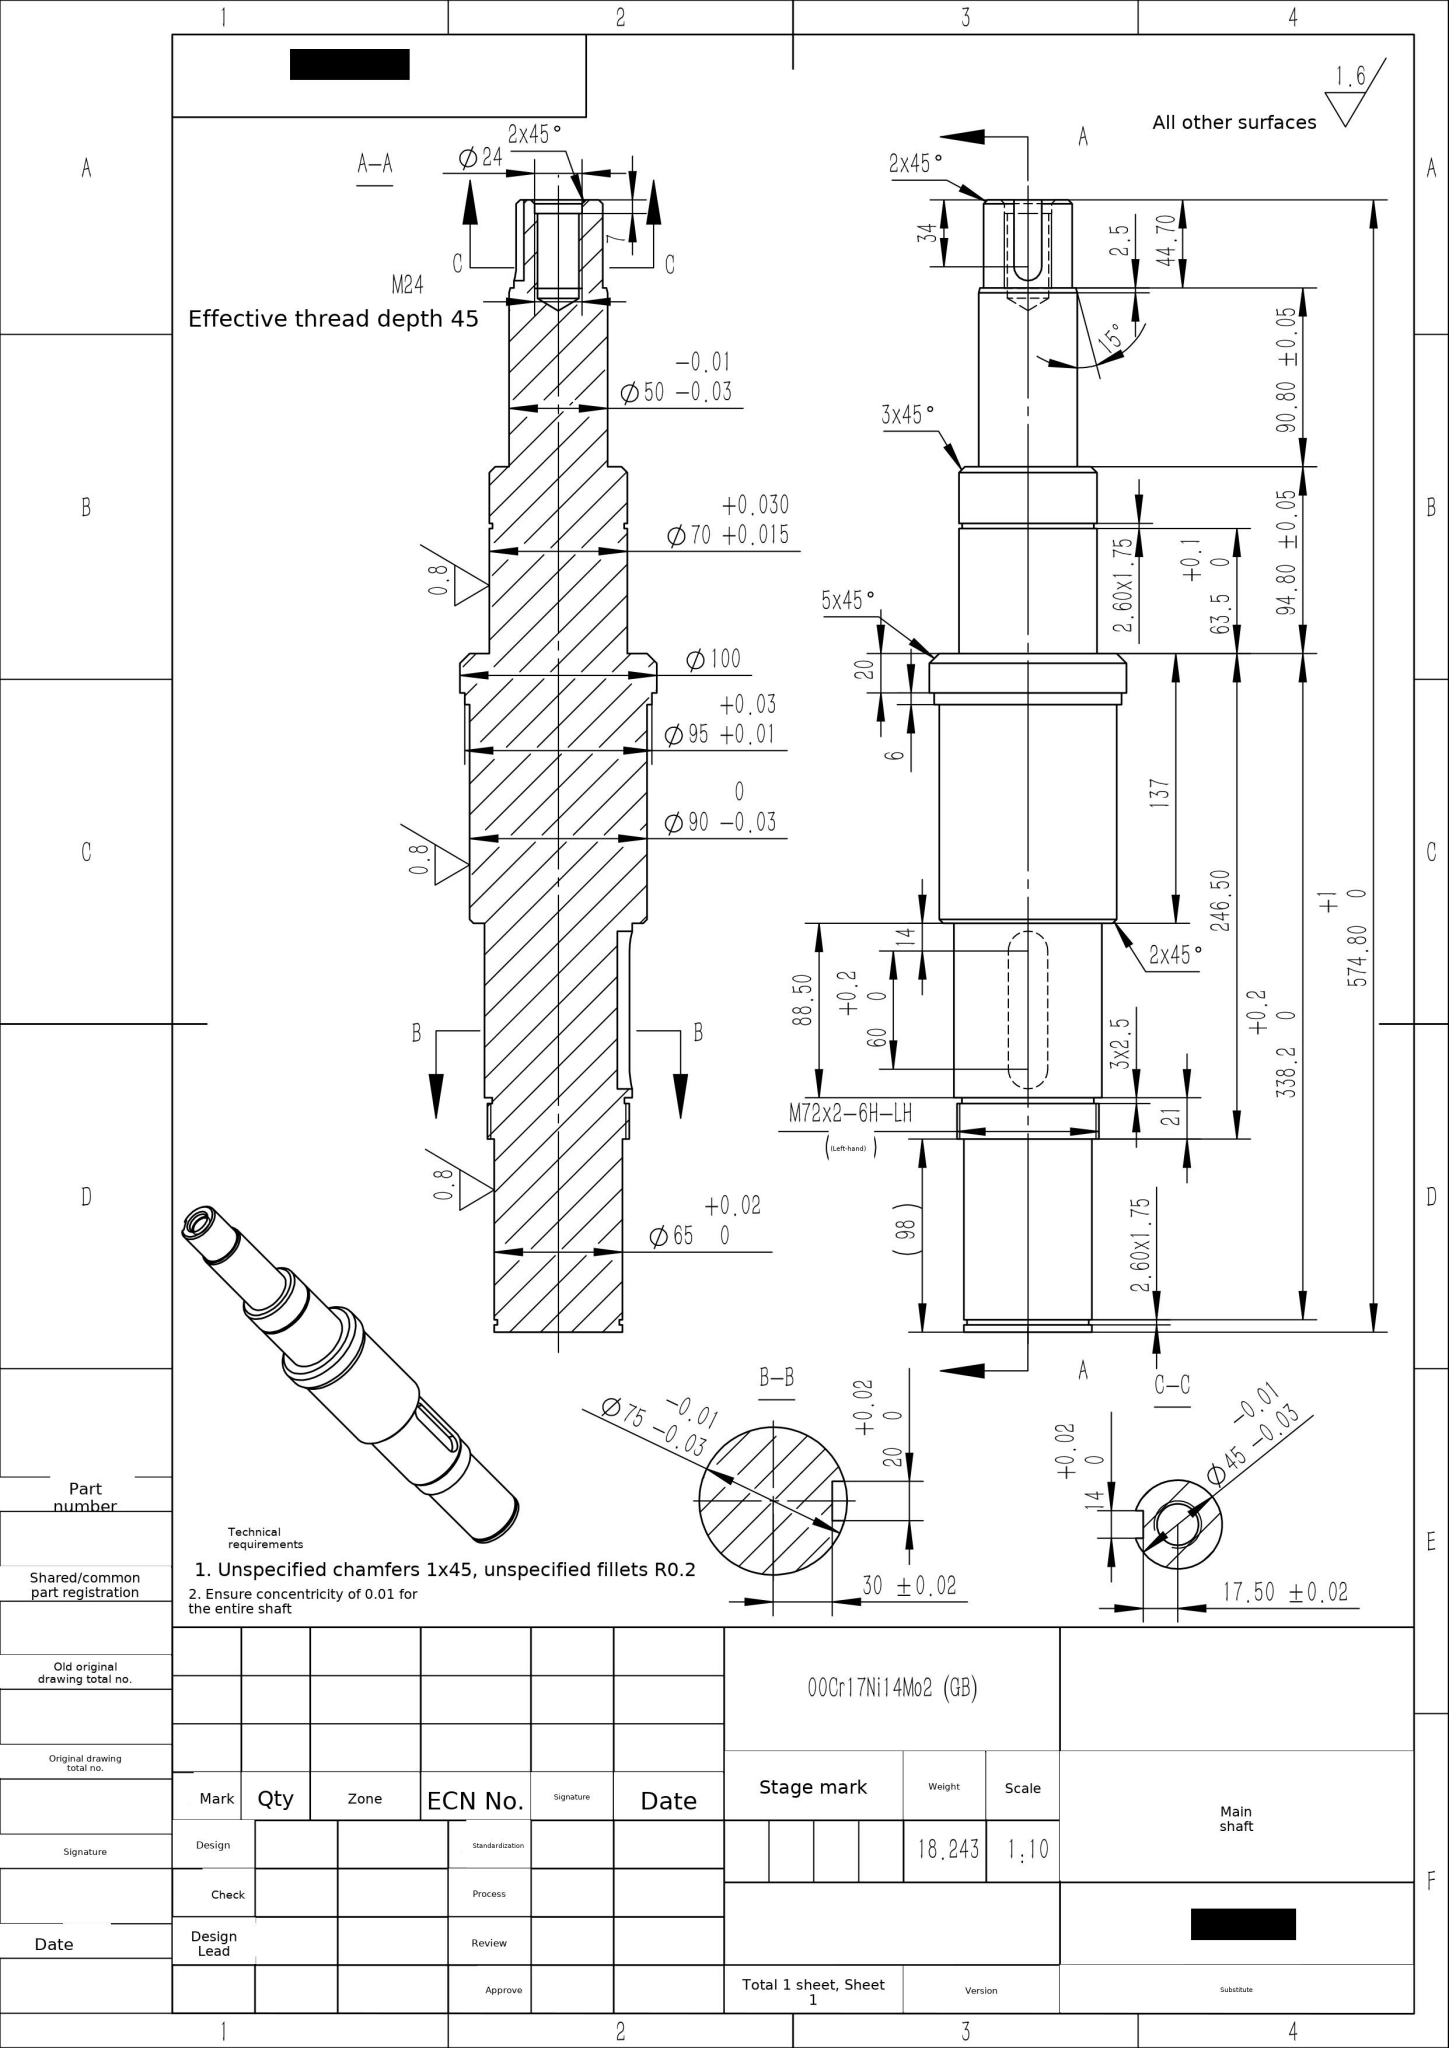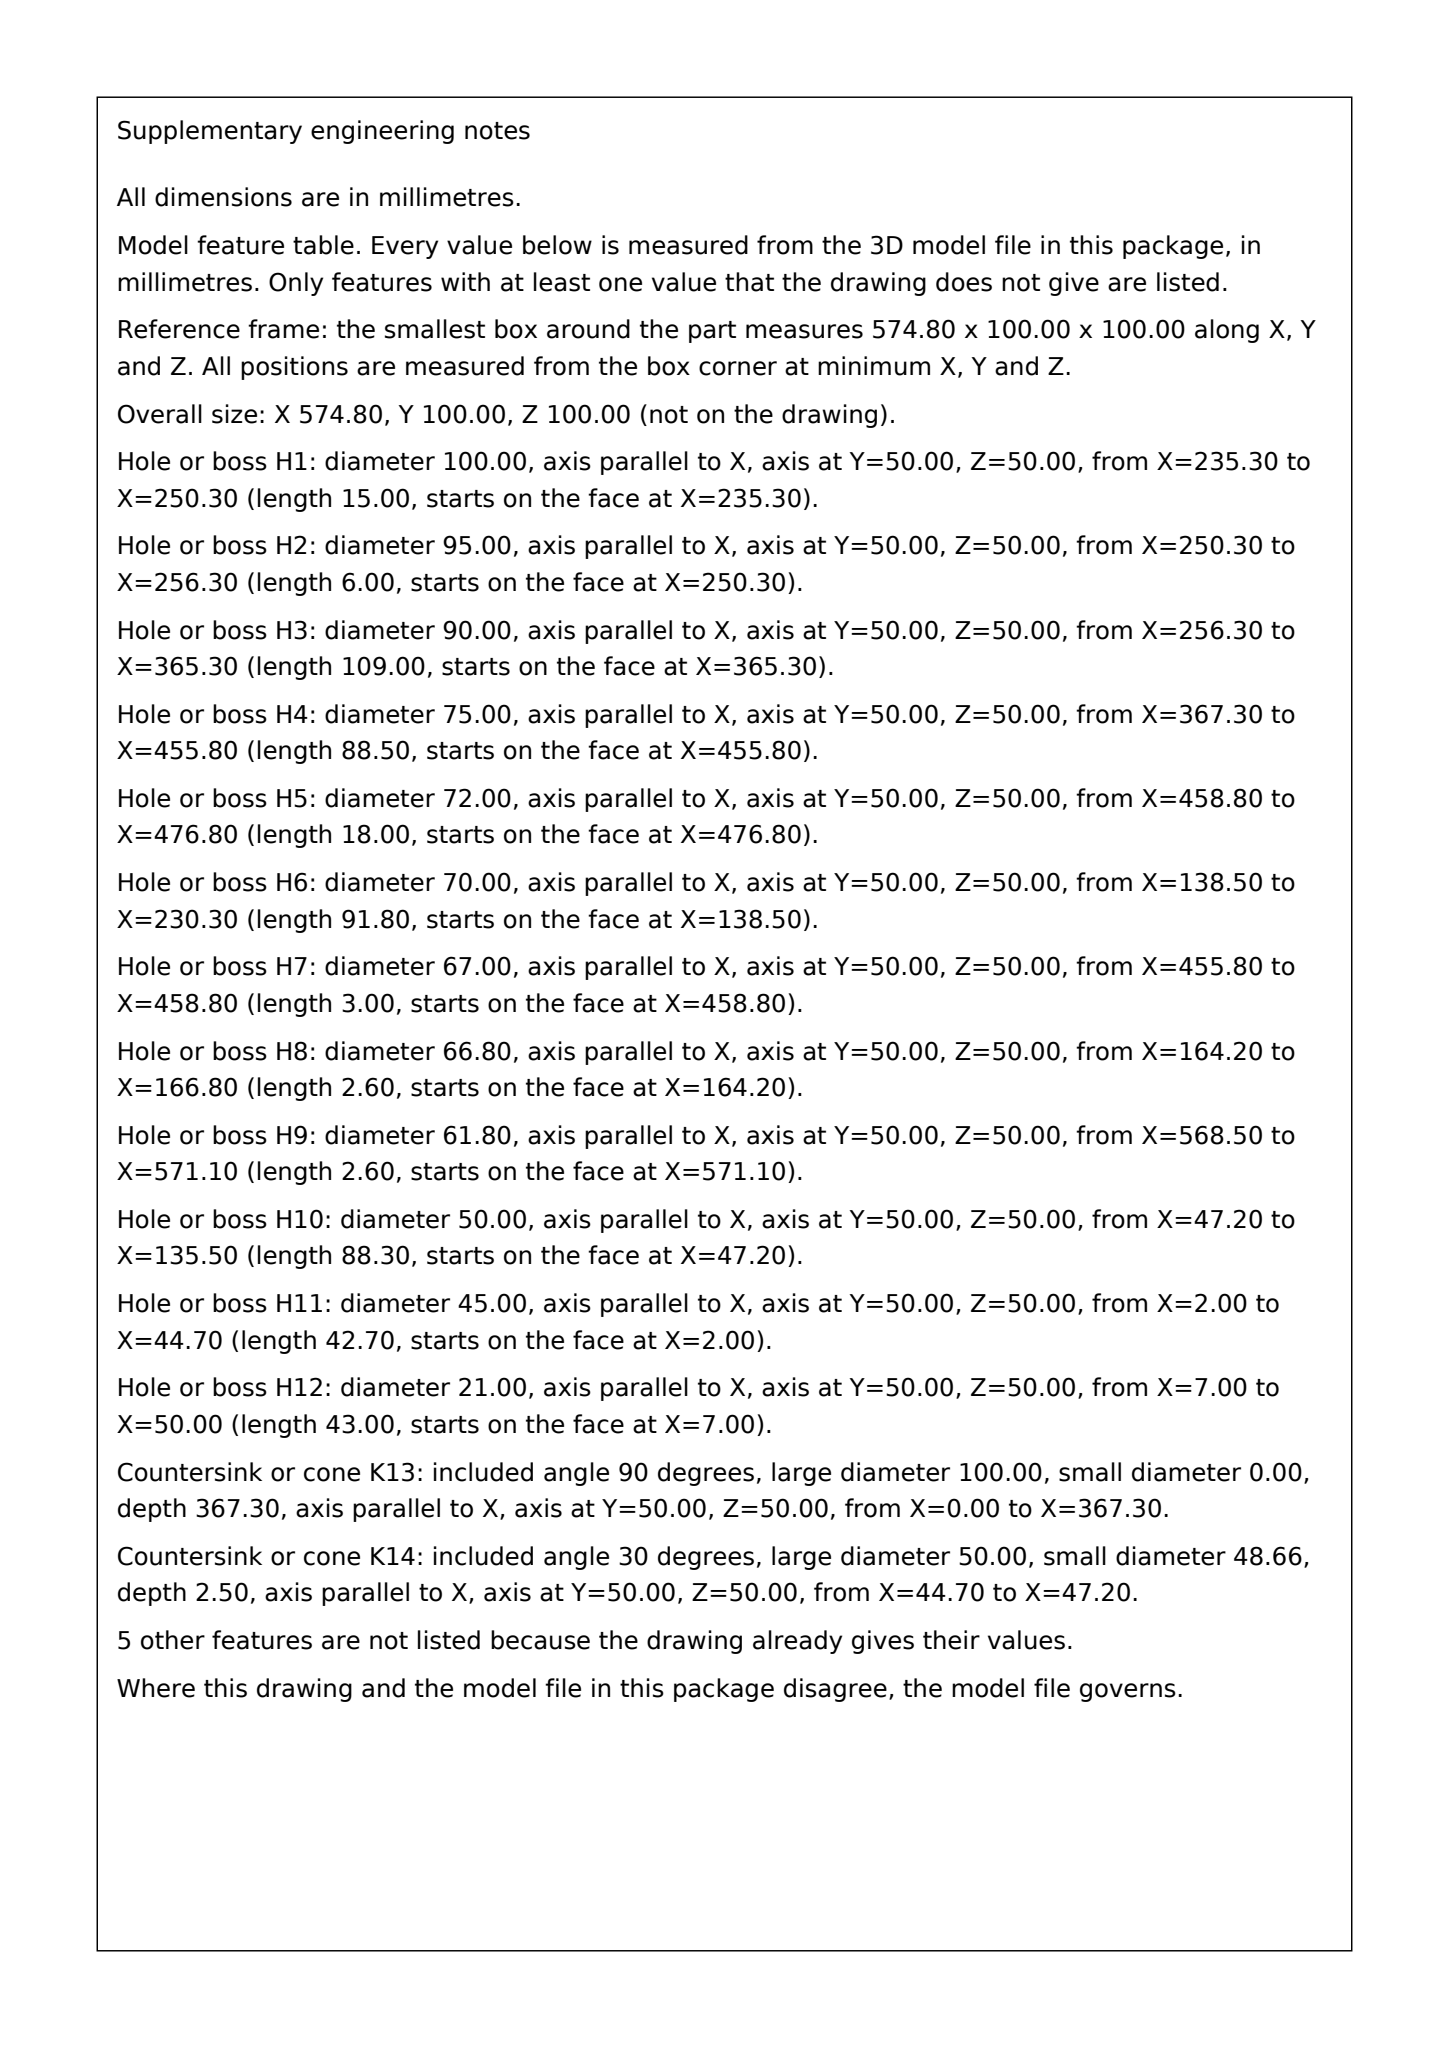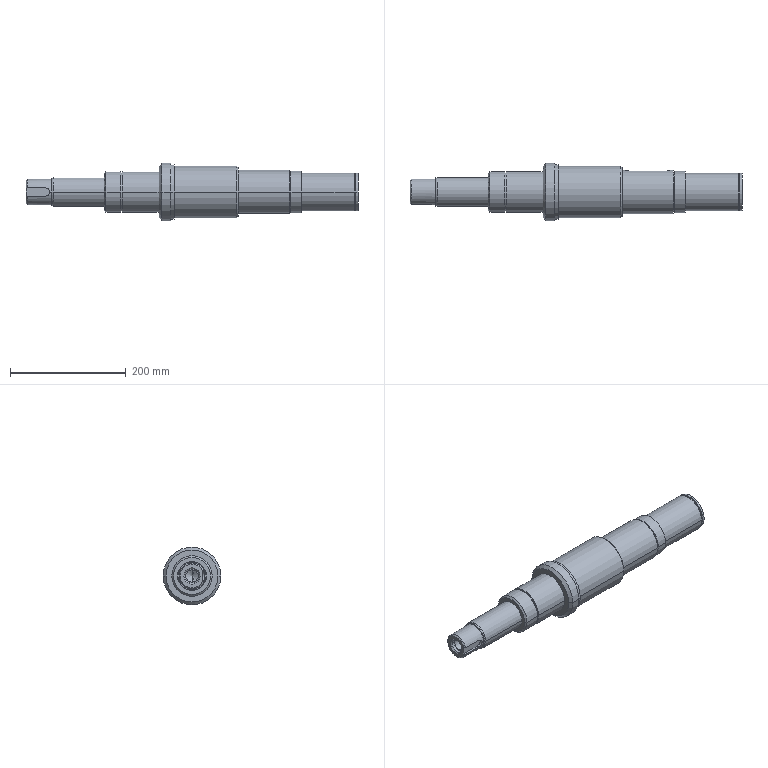Part | SolidWorks | mm | material 00Cr17Ni14Mo2 (GB) | 1 solid | 71 faces | box 574.8 x 100 x 100 mm | volume 2280370 mm3 | cylinder 35 | plane 22 | cone 14 | commonest cylinder face diameters 65 x4 70 x4 21 x2 24 x2 61.8 x2 72 x2 67 x2 90 x2
build123d program:
from build123d import *

# Parameters (mm, degrees)
CHAMFER1_SIZE          = 3
SKETCH6_W              = 14
SKETCH6_H              = 7.479
CUT_EXTRUDE4_DEPTH     = 34
SKETCH8_R              = 12
CUT_EXTRUDE6_DEPTH     = 7
M24_TAPPED_HOLE1_D     = 21
M24_TAPPED_HOLE1_DEPTH = 43
M24_TAPPED_HOLE1_TIP   = 6.309
CHAMFER3_SIZE          = 2
CHAMFER4_SIZE          = 2
CHAMFER5_SIZE          = 2.5
CHAMFER5_SIZE2         = 0.6699
SKETCH16_R             = 7
CUT_EXTRUDE9_DEPTH     = 18
CHAMFER7_SIZE          = 5
CUT_EXTRUDE10_START    = 30
CUT_EXTRUDE10_DEPTH    = 550.133
CHAMFER8_SIZE          = 2


with BuildPart() as part:
    # Sketch1 → Revolve1 (revolve)
    with BuildSketch(Plane.XY, mode=Mode.PRIVATE) as revolve1_sk:
        Polygon((0, 0), (0, 22.5), (44.7, 22.5), (44.7, 25), (135.5, 25), (135.5, 35), (164.2, 35), (164.2, 33.4), (166.8, 33.4), (166.8, 35), (230.3, 35), (230.3, 50), (250.3, 50), (250.3, 47.5), (256.3, 47.5), (256.3, 45), (367.3, 45), (367.3, 37.5), (455.8, 37.5), (455.8, 33.5), (458.8, 33.5), (458.8, 36), (476.8, 36), (476.8, 32.5), (568.5, 32.5), (568.5, 30.9), (571.1, 30.9), (571.1, 32.5), (574.8, 32.5), (574.8, 0), align=None)
    revolve(revolve1_sk.sketch.rotate(Axis((0, 0, 0), (1, 0, 0)), 180), axis=Axis((0, 0, 0), (1, 0, 0)))

    # Chamfer1
    chamfer1_edges = [part.edges().sort_by_distance(p)[0] for p in [
        (135.5, 35, 0),
    ]]
    chamfer(chamfer1_edges, length=CHAMFER1_SIZE)

    # Sketch6 → Cut-Extrude4 (cut)
    with BuildSketch(Plane(origin=(0, 0, 0), x_dir=(0, 0, -1), z_dir=(1, 0, 0))):
        with Locations((0, -21.24)):
            Rectangle(SKETCH6_W, SKETCH6_H)
    extrude(amount=CUT_EXTRUDE4_DEPTH, mode=Mode.SUBTRACT)

    # Sketch8 → Cut-Extrude6 (cut)
    with BuildSketch(Plane.ZY):
        with Locations(Location((0, 0, 0), (0, 0, 270))):
            Circle(SKETCH8_R)
    extrude(amount=-CUT_EXTRUDE6_DEPTH, mode=Mode.SUBTRACT)

    # M24 Tapped Hole1
    with Locations(Plane(origin=(7, 0, 0), x_dir=(0, -1, 0), z_dir=(-1, 0, 0))):
        with Locations((0, 0)):
            Hole(M24_TAPPED_HOLE1_D / 2, depth=M24_TAPPED_HOLE1_DEPTH)
            with Locations((0, 0, -(M24_TAPPED_HOLE1_DEPTH + M24_TAPPED_HOLE1_TIP / 2))):  # 118° drill point
                Cone(0, M24_TAPPED_HOLE1_D / 2, M24_TAPPED_HOLE1_TIP, mode=Mode.SUBTRACT)

    # Chamfer3
    chamfer3_edges = [part.edges().sort_by_distance(p)[0] for p in [
        (0, 12, 0),
    ]]
    chamfer(chamfer3_edges, length=CHAMFER3_SIZE)

    # Chamfer4
    chamfer4_edges = [part.edges().sort_by_distance(p)[0] for p in [
        (0, 22.5, 0),
    ]]
    chamfer(chamfer4_edges, length=CHAMFER4_SIZE)

    # Chamfer5
    chamfer5_edges = [part.edges().sort_by_distance(p)[0] for p in [
        (44.7, 25, 0),
    ]]
    chamfer5_side = [part.faces().sort_by_distance(p)[0] for p in [
        (90.1, 25, 0),
    ]]
    chamfer(chamfer5_edges, length=CHAMFER5_SIZE, length2=CHAMFER5_SIZE2, reference=chamfer5_side[0])

    # Sketch16 → Cut-Extrude9 (cut)
    with BuildSketch(Plane(origin=(0, -17.5, 0), x_dir=(-1, 0, 0), z_dir=(0, -1, 0))):
        with Locations((-34, 0)):
            Circle(SKETCH16_R)
    extrude(amount=CUT_EXTRUDE9_DEPTH, mode=Mode.SUBTRACT)

    # Chamfer7
    chamfer7_edges = [part.edges().sort_by_distance(p)[0] for p in [
        (230.3, 50, 0),
    ]]
    chamfer(chamfer7_edges, length=CHAMFER7_SIZE)

    # Sketch18 → Cut-Extrude10 (cut, through all)
    with BuildSketch(Plane(origin=(0, 0, 0), x_dir=(1, 0, 0), z_dir=(0, 1, 0)).offset(CUT_EXTRUDE10_START)):
        with BuildLine():
            Line((381.3, 10), (441.3, 10))
            ThreePointArc((441.3, 10), (451.3, 0), (441.3, -10))
            Line((441.3, -10), (381.3, -10))
            ThreePointArc((381.3, -10), (371.3, 0), (381.3, 10))
        make_face()
    extrude(amount=CUT_EXTRUDE10_DEPTH, mode=Mode.SUBTRACT)

    # Chamfer8
    chamfer8_edges = [part.edges().sort_by_distance(p)[0] for p in [
        (367.3, 45, 0),
    ]]
    chamfer(chamfer8_edges, length=CHAMFER8_SIZE)


solid = part.part